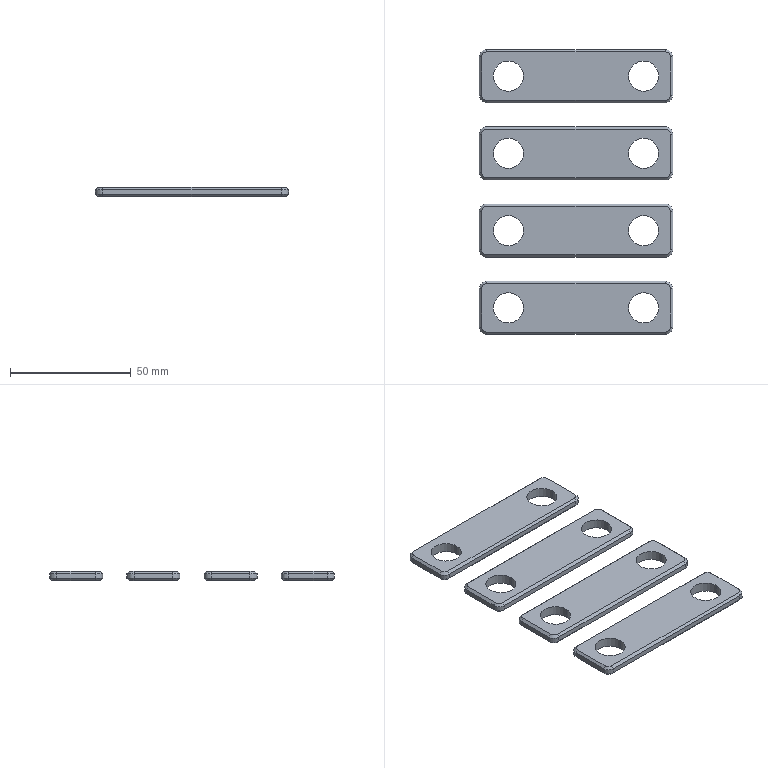CAM job | Mastercam | mm | 8 operations | part box 80 x 118 x 4
1. 2D High Speed (2D Area Mill) | 4 - 4 平铣刀
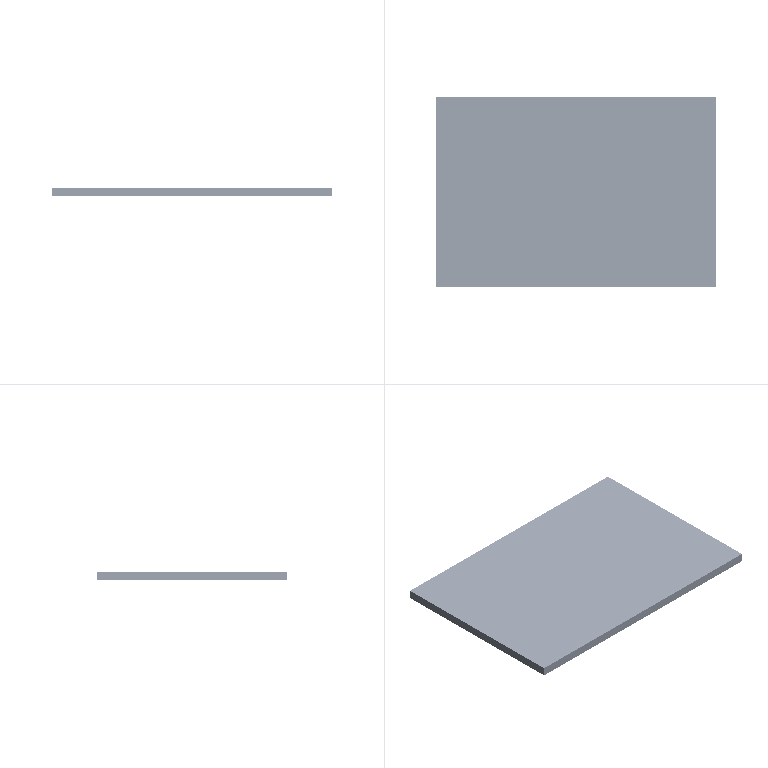2. Contour (Ramp) | 2 - 2 平铣刀
3. Contour (Ramp) | 2 - 2 平铣刀
4. Contour (Ramp) | 2 - 2 平铣刀
5. Contour (2D chamfer) | 7 - 4 倒角刀
6. Contour (2D chamfer) | 7 - 4 倒角刀
7. Contour (2D chamfer) | 7 - 4 倒角刀
8. Contour (2D chamfer) | 7 - 4 倒角刀